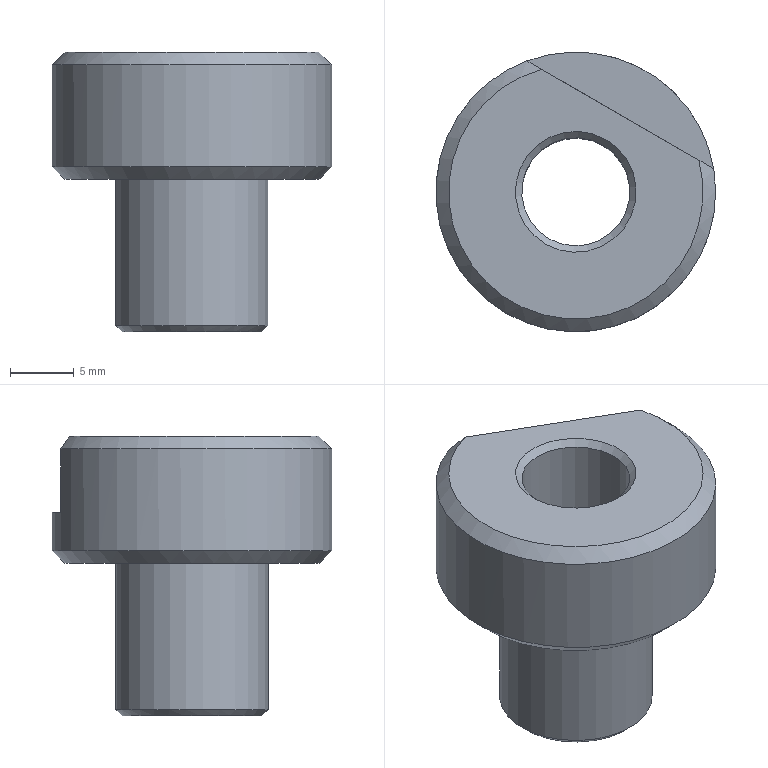Component | NX | DRILL_BUSH_5 | 1 solid | 13 faces | box 22 x 22 x 22 mm | volume 3557 mm3 | plane 5 | cone 5 | cylinder 3 | commonest cylinder face diameters 12 x1 22 x1 8.5 x1
STEP:
#1=CARTESIAN_POINT('',(0.,0.,0.));
#2=DIRECTION('',(0.,0.,1.));
#3=DIRECTION('',(1.,0.,0.));
#4=AXIS2_PLACEMENT_3D('',#1,#2,#3);
#5=CARTESIAN_POINT('',(-32.75,-56.725,158.));
#6=VERTEX_POINT('',#5);
#7=CARTESIAN_POINT('',(-30.,-51.962,158.));
#8=DIRECTION('',(0.,0.,-1.));
#9=DIRECTION('',(-0.5,-0.866,0.));
#10=AXIS2_PLACEMENT_3D('',#7,#8,#9);
#11=CIRCLE('',#10,5.5);
#12=CARTESIAN_POINT('',(-30.,-51.962,158.));
#13=DIRECTION('',(0.,0.,-1.));
#14=DIRECTION('',(-0.5,-0.866,0.));
#15=AXIS2_PLACEMENT_3D('',#12,#13,#14);
#16=PLANE('',#15);
#17=CARTESIAN_POINT('',(0.,0.));
#18=DIRECTION('',(1.,0.));
#19=AXIS2_PLACEMENT_2D('',#17,#18);
#20=CIRCLE('',#19,5.5);
#21=(GEOMETRIC_REPRESENTATION_CONTEXT(2)PARAMETRIC_REPRESENTATION_CONTEXT()REPRESENTATION_CONTEXT('',''));
#22=DEFINITIONAL_REPRESENTATION('',(#20),#21);
#23=PCURVE('',#16,#22);
#24=CARTESIAN_POINT('',(-30.,-51.962,158.5));
#25=DIRECTION('',(0.,0.,1.));
#26=DIRECTION('',(0.5,0.866,0.));
#27=AXIS2_PLACEMENT_3D('',#24,#25,#26);
#28=CONICAL_SURFACE('',#27,6.,0.7854);
#29=CARTESIAN_POINT('',(9.425,-0.5));
#30=DIRECTION('',(-1.,0.));
#31=VECTOR('',#30,1.);
#32=LINE('',#29,#31);
#33=(GEOMETRIC_REPRESENTATION_CONTEXT(2)PARAMETRIC_REPRESENTATION_CONTEXT()REPRESENTATION_CONTEXT('',''));
#34=DEFINITIONAL_REPRESENTATION('',(#32),#33);
#35=PCURVE('',#28,#34);
#36=SURFACE_CURVE('',#11,(#23,#35),.PCURVE_S1.);
#37=EDGE_CURVE('',#6,#6,#36,.T.);
#38=ORIENTED_EDGE('',*,*,#37,.T.);
#39=EDGE_LOOP('',(#38));
#40=FACE_BOUND('',#39,.T.);
#41=CARTESIAN_POINT('',(-32.375,-56.075,158.));
#42=VERTEX_POINT('',#41);
#43=CARTESIAN_POINT('',(-30.,-51.962,158.));
#44=DIRECTION('',(0.,0.,1.));
#45=DIRECTION('',(-0.5,-0.866,0.));
#46=AXIS2_PLACEMENT_3D('',#43,#44,#45);
#47=CIRCLE('',#46,4.75);
#48=CARTESIAN_POINT('',(4.75,0.));
#49=CARTESIAN_POINT('',(4.75,-8.227));
#50=CARTESIAN_POINT('',(-2.375,-4.114));
#51=CARTESIAN_POINT('',(-9.5,-0.));
#52=CARTESIAN_POINT('',(-2.375,4.114));
#53=CARTESIAN_POINT('',(4.75,8.227));
#54=CARTESIAN_POINT('',(4.75,0.));
#55=(BOUNDED_CURVE()B_SPLINE_CURVE(2,(#48,#49,#50,#51,#52,#53,#54),.UNSPECIFIED.,.T.,.F.)B_SPLINE_CURVE_WITH_KNOTS((1,2,2,2,2,1),(-2.094,0.,2.094,4.189,6.283,8.378),.UNSPECIFIED.)CURVE()GEOMETRIC_REPRESENTATION_ITEM()RATIONAL_B_SPLINE_CURVE((1.,0.5,1.,0.5,1.,0.5,1.))REPRESENTATION_ITEM(''));
#56=(GEOMETRIC_REPRESENTATION_CONTEXT(2)PARAMETRIC_REPRESENTATION_CONTEXT()REPRESENTATION_CONTEXT('',''));
#57=DEFINITIONAL_REPRESENTATION('',(#55),#56);
#58=PCURVE('',#16,#57);
#59=CARTESIAN_POINT('',(-30.,-51.962,158.5));
#60=DIRECTION('',(0.,0.,-1.));
#61=DIRECTION('',(-0.5,-0.866,0.));
#62=AXIS2_PLACEMENT_3D('',#59,#60,#61);
#63=CONICAL_SURFACE('',#62,4.25,0.7854);
#64=CARTESIAN_POINT('',(6.283,0.5));
#65=DIRECTION('',(-1.,0.));
#66=VECTOR('',#65,1.);
#67=LINE('',#64,#66);
#68=(GEOMETRIC_REPRESENTATION_CONTEXT(2)PARAMETRIC_REPRESENTATION_CONTEXT()REPRESENTATION_CONTEXT('',''));
#69=DEFINITIONAL_REPRESENTATION('',(#67),#68);
#70=PCURVE('',#63,#69);
#71=SURFACE_CURVE('',#47,(#58,#70),.PCURVE_S1.);
#72=EDGE_CURVE('',#42,#42,#71,.T.);
#73=ORIENTED_EDGE('',*,*,#72,.T.);
#74=EDGE_LOOP('',(#73));
#75=FACE_BOUND('',#74,.T.);
#76=ADVANCED_FACE('',(#40,#75),#16,.T.);
#77=CARTESIAN_POINT('',(-33.,-57.158,158.5));
#78=VERTEX_POINT('',#77);
#79=CARTESIAN_POINT('',(-30.,-51.962,158.5));
#80=DIRECTION('',(0.,0.,1.));
#81=DIRECTION('',(-0.5,-0.866,0.));
#82=AXIS2_PLACEMENT_3D('',#79,#80,#81);
#83=CIRCLE('',#82,6.);
#84=CARTESIAN_POINT('',(-30.,-51.962,158.));
#85=DIRECTION('',(0.,0.,1.));
#86=DIRECTION('',(0.5,0.866,0.));
#87=AXIS2_PLACEMENT_3D('',#84,#85,#86);
#88=CYLINDRICAL_SURFACE('',#87,6.);
#89=CARTESIAN_POINT('',(3.142,0.5));
#90=DIRECTION('',(1.,0.));
#91=VECTOR('',#90,1.);
#92=LINE('',#89,#91);
#93=(GEOMETRIC_REPRESENTATION_CONTEXT(2)PARAMETRIC_REPRESENTATION_CONTEXT()REPRESENTATION_CONTEXT('',''));
#94=DEFINITIONAL_REPRESENTATION('',(#92),#93);
#95=PCURVE('',#88,#94);
#96=CARTESIAN_POINT('',(3.142,-0.));
#97=DIRECTION('',(1.,0.));
#98=VECTOR('',#97,1.);
#99=LINE('',#96,#98);
#100=(GEOMETRIC_REPRESENTATION_CONTEXT(2)PARAMETRIC_REPRESENTATION_CONTEXT()REPRESENTATION_CONTEXT('',''));
#101=DEFINITIONAL_REPRESENTATION('',(#99),#100);
#102=PCURVE('',#28,#101);
#103=SURFACE_CURVE('',#83,(#95,#102),.PCURVE_S1.);
#104=EDGE_CURVE('',#78,#78,#103,.T.);
#105=ORIENTED_EDGE('',*,*,#104,.T.);
#106=CARTESIAN_POINT('',(-33.,-57.158,170.));
#107=VERTEX_POINT('',#106);
#108=CARTESIAN_POINT('',(-33.,-57.158,158.5));
#109=CARTESIAN_POINT('',(-33.,-57.158,170.));
#110=B_SPLINE_CURVE_WITH_KNOTS('',1,(#108,#109),.UNSPECIFIED.,.F.,.F.,(2,2),(0.5,12.),.PIECEWISE_BEZIER_KNOTS.);
#111=CARTESIAN_POINT('',(9.425,0.));
#112=DIRECTION('',(0.,1.));
#113=VECTOR('',#112,1.);
#114=LINE('',#111,#113);
#115=(GEOMETRIC_REPRESENTATION_CONTEXT(2)PARAMETRIC_REPRESENTATION_CONTEXT()REPRESENTATION_CONTEXT('',''));
#116=DEFINITIONAL_REPRESENTATION('',(#114),#115);
#117=PCURVE('',#88,#116);
#118=CARTESIAN_POINT('',(3.142,0.));
#119=DIRECTION('',(0.,1.));
#120=VECTOR('',#119,1.);
#121=LINE('',#118,#120);
#122=(GEOMETRIC_REPRESENTATION_CONTEXT(2)PARAMETRIC_REPRESENTATION_CONTEXT()REPRESENTATION_CONTEXT('',''));
#123=DEFINITIONAL_REPRESENTATION('',(#121),#122);
#124=PCURVE('',#88,#123);
#125=SEAM_CURVE('',#110,(#117,#124),.PCURVE_S1.);
#126=EDGE_CURVE('',#78,#107,#125,.T.);
#127=ORIENTED_EDGE('',*,*,#126,.T.);
#128=CARTESIAN_POINT('',(-30.,-51.962,170.));
#129=DIRECTION('',(0.,0.,1.));
#130=DIRECTION('',(-0.5,-0.866,0.));
#131=AXIS2_PLACEMENT_3D('',#128,#129,#130);
#132=CIRCLE('',#131,6.);
#133=CARTESIAN_POINT('',(3.142,12.));
#134=DIRECTION('',(1.,0.));
#135=VECTOR('',#134,1.);
#136=LINE('',#133,#135);
#137=(GEOMETRIC_REPRESENTATION_CONTEXT(2)PARAMETRIC_REPRESENTATION_CONTEXT()REPRESENTATION_CONTEXT('',''));
#138=DEFINITIONAL_REPRESENTATION('',(#136),#137);
#139=PCURVE('',#88,#138);
#140=CARTESIAN_POINT('',(-30.,-51.962,170.));
#141=DIRECTION('',(0.,0.,-1.));
#142=DIRECTION('',(-0.5,-0.866,0.));
#143=AXIS2_PLACEMENT_3D('',#140,#141,#142);
#144=PLANE('',#143);
#145=CARTESIAN_POINT('',(6.,0.));
#146=CARTESIAN_POINT('',(6.,-10.392));
#147=CARTESIAN_POINT('',(-3.,-5.196));
#148=CARTESIAN_POINT('',(-12.,-0.));
#149=CARTESIAN_POINT('',(-3.,5.196));
#150=CARTESIAN_POINT('',(6.,10.392));
#151=CARTESIAN_POINT('',(6.,0.));
#152=(BOUNDED_CURVE()B_SPLINE_CURVE(2,(#145,#146,#147,#148,#149,#150,#151),.UNSPECIFIED.,.T.,.F.)B_SPLINE_CURVE_WITH_KNOTS((1,2,2,2,2,1),(-2.094,0.,2.094,4.189,6.283,8.378),.UNSPECIFIED.)CURVE()GEOMETRIC_REPRESENTATION_ITEM()RATIONAL_B_SPLINE_CURVE((1.,0.5,1.,0.5,1.,0.5,1.))REPRESENTATION_ITEM(''));
#153=(GEOMETRIC_REPRESENTATION_CONTEXT(2)PARAMETRIC_REPRESENTATION_CONTEXT()REPRESENTATION_CONTEXT('',''));
#154=DEFINITIONAL_REPRESENTATION('',(#152),#153);
#155=PCURVE('',#144,#154);
#156=SURFACE_CURVE('',#132,(#139,#155),.PCURVE_S1.);
#157=EDGE_CURVE('',#107,#107,#156,.T.);
#158=ORIENTED_EDGE('',*,*,#157,.F.);
#159=ORIENTED_EDGE('',*,*,#126,.F.);
#160=EDGE_LOOP('',(#105,#127,#158,#159));
#161=FACE_BOUND('',#160,.T.);
#162=ADVANCED_FACE('',(#161),#88,.T.);
#163=CARTESIAN_POINT('',(-27.625,-47.848,180.));
#164=VERTEX_POINT('',#163);
#165=CARTESIAN_POINT('',(-30.,-51.962,180.));
#166=DIRECTION('',(0.,0.,-1.));
#167=DIRECTION('',(0.5,0.866,0.));
#168=AXIS2_PLACEMENT_3D('',#165,#166,#167);
#169=CIRCLE('',#168,4.75);
#170=CARTESIAN_POINT('',(-30.,-51.962,180.));
#171=DIRECTION('',(0.,0.,1.));
#172=DIRECTION('',(0.5,0.866,0.));
#173=AXIS2_PLACEMENT_3D('',#170,#171,#172);
#174=PLANE('',#173);
#175=CARTESIAN_POINT('',(4.75,0.));
#176=CARTESIAN_POINT('',(4.75,-8.227));
#177=CARTESIAN_POINT('',(-2.375,-4.114));
#178=CARTESIAN_POINT('',(-9.5,-0.));
#179=CARTESIAN_POINT('',(-2.375,4.114));
#180=CARTESIAN_POINT('',(4.75,8.227));
#181=CARTESIAN_POINT('',(4.75,0.));
#182=(BOUNDED_CURVE()B_SPLINE_CURVE(2,(#175,#176,#177,#178,#179,#180,#181),.UNSPECIFIED.,.T.,.F.)B_SPLINE_CURVE_WITH_KNOTS((1,2,2,2,2,1),(-2.094,0.,2.094,4.189,6.283,8.378),.UNSPECIFIED.)CURVE()GEOMETRIC_REPRESENTATION_ITEM()RATIONAL_B_SPLINE_CURVE((1.,0.5,1.,0.5,1.,0.5,1.))REPRESENTATION_ITEM(''));
#183=(GEOMETRIC_REPRESENTATION_CONTEXT(2)PARAMETRIC_REPRESENTATION_CONTEXT()REPRESENTATION_CONTEXT('',''));
#184=DEFINITIONAL_REPRESENTATION('',(#182),#183);
#185=PCURVE('',#174,#184);
#186=CARTESIAN_POINT('',(-30.,-51.962,180.));
#187=DIRECTION('',(0.,0.,1.));
#188=DIRECTION('',(0.5,0.866,0.));
#189=AXIS2_PLACEMENT_3D('',#186,#187,#188);
#190=CONICAL_SURFACE('',#189,4.75,0.7854);
#191=CARTESIAN_POINT('',(6.283,0.));
#192=DIRECTION('',(-1.,0.));
#193=VECTOR('',#192,1.);
#194=LINE('',#191,#193);
#195=(GEOMETRIC_REPRESENTATION_CONTEXT(2)PARAMETRIC_REPRESENTATION_CONTEXT()REPRESENTATION_CONTEXT('',''));
#196=DEFINITIONAL_REPRESENTATION('',(#194),#195);
#197=PCURVE('',#190,#196);
#198=SURFACE_CURVE('',#169,(#185,#197),.PCURVE_S1.);
#199=EDGE_CURVE('',#164,#164,#198,.T.);
#200=ORIENTED_EDGE('',*,*,#199,.T.);
#201=EDGE_LOOP('',(#200));
#202=FACE_BOUND('',#201,.T.);
#203=CARTESIAN_POINT('',(-32.685,-42.329,180.));
#204=VERTEX_POINT('',#203);
#205=CARTESIAN_POINT('',(-20.315,-49.47,180.));
#206=VERTEX_POINT('',#205);
#207=CARTESIAN_POINT('',(-37.758,-39.399,180.));
#208=DIRECTION('',(0.866,-0.5,0.));
#209=VECTOR('',#208,1.);
#210=LINE('',#207,#209);
#211=CARTESIAN_POINT('',(7.,13.));
#212=DIRECTION('',(0.,-1.));
#213=VECTOR('',#212,1.);
#214=LINE('',#211,#213);
#215=(GEOMETRIC_REPRESENTATION_CONTEXT(2)PARAMETRIC_REPRESENTATION_CONTEXT()REPRESENTATION_CONTEXT('',''));
#216=DEFINITIONAL_REPRESENTATION('',(#214),#215);
#217=PCURVE('',#174,#216);
#218=CARTESIAN_POINT('',(-37.758,-39.399,174.));
#219=DIRECTION('',(-0.5,-0.866,0.));
#220=DIRECTION('',(0.866,-0.5,0.));
#221=AXIS2_PLACEMENT_3D('',#218,#219,#220);
#222=PLANE('',#221);
#223=CARTESIAN_POINT('',(0.,6.));
#224=DIRECTION('',(1.,0.));
#225=VECTOR('',#224,1.);
#226=LINE('',#223,#225);
#227=(GEOMETRIC_REPRESENTATION_CONTEXT(2)PARAMETRIC_REPRESENTATION_CONTEXT()REPRESENTATION_CONTEXT('',''));
#228=DEFINITIONAL_REPRESENTATION('',(#226),#227);
#229=PCURVE('',#222,#228);
#230=SURFACE_CURVE('',#210,(#217,#229),.PCURVE_S1.);
#231=EDGE_CURVE('',#204,#206,#230,.T.);
#232=ORIENTED_EDGE('',*,*,#231,.F.);
#233=CARTESIAN_POINT('',(-30.,-51.962,180.));
#234=DIRECTION('',(0.,0.,1.));
#235=DIRECTION('',(0.5,0.866,0.));
#236=AXIS2_PLACEMENT_3D('',#233,#234,#235);
#237=CIRCLE('',#236,10.);
#238=CARTESIAN_POINT('',(0.,0.));
#239=DIRECTION('',(1.,0.));
#240=AXIS2_PLACEMENT_2D('',#238,#239);
#241=CIRCLE('',#240,10.);
#242=(GEOMETRIC_REPRESENTATION_CONTEXT(2)PARAMETRIC_REPRESENTATION_CONTEXT()REPRESENTATION_CONTEXT('',''));
#243=DEFINITIONAL_REPRESENTATION('',(#241),#242);
#244=PCURVE('',#174,#243);
#245=CARTESIAN_POINT('',(-30.,-51.962,179.));
#246=DIRECTION('',(0.,0.,-1.));
#247=DIRECTION('',(-0.5,-0.866,0.));
#248=AXIS2_PLACEMENT_3D('',#245,#246,#247);
#249=CONICAL_SURFACE('',#248,11.,0.7854);
#250=CARTESIAN_POINT('',(3.142,-1.));
#251=DIRECTION('',(-1.,0.));
#252=VECTOR('',#251,1.);
#253=LINE('',#250,#252);
#254=(GEOMETRIC_REPRESENTATION_CONTEXT(2)PARAMETRIC_REPRESENTATION_CONTEXT()REPRESENTATION_CONTEXT('',''));
#255=DEFINITIONAL_REPRESENTATION('',(#253),#254);
#256=PCURVE('',#249,#255);
#257=SURFACE_CURVE('',#237,(#244,#256),.PCURVE_S1.);
#258=EDGE_CURVE('',#204,#206,#257,.T.);
#259=ORIENTED_EDGE('',*,*,#258,.T.);
#260=EDGE_LOOP('',(#232,#259));
#261=FACE_BOUND('',#260,.T.);
#262=ADVANCED_FACE('',(#202,#261),#174,.T.);
#263=CARTESIAN_POINT('',(-35.,-60.622,170.));
#264=VERTEX_POINT('',#263);
#265=CARTESIAN_POINT('',(-30.,-51.962,170.));
#266=DIRECTION('',(0.,0.,-1.));
#267=DIRECTION('',(-0.5,-0.866,0.));
#268=AXIS2_PLACEMENT_3D('',#265,#266,#267);
#269=CIRCLE('',#268,10.);
#270=CARTESIAN_POINT('',(0.,0.));
#271=DIRECTION('',(1.,0.));
#272=AXIS2_PLACEMENT_2D('',#270,#271);
#273=CIRCLE('',#272,10.);
#274=(GEOMETRIC_REPRESENTATION_CONTEXT(2)PARAMETRIC_REPRESENTATION_CONTEXT()REPRESENTATION_CONTEXT('',''));
#275=DEFINITIONAL_REPRESENTATION('',(#273),#274);
#276=PCURVE('',#144,#275);
#277=CARTESIAN_POINT('',(-30.,-51.962,171.));
#278=DIRECTION('',(0.,0.,1.));
#279=DIRECTION('',(0.5,0.866,0.));
#280=AXIS2_PLACEMENT_3D('',#277,#278,#279);
#281=CONICAL_SURFACE('',#280,11.,0.7854);
#282=CARTESIAN_POINT('',(9.425,-1.));
#283=DIRECTION('',(-1.,0.));
#284=VECTOR('',#283,1.);
#285=LINE('',#282,#284);
#286=(GEOMETRIC_REPRESENTATION_CONTEXT(2)PARAMETRIC_REPRESENTATION_CONTEXT()REPRESENTATION_CONTEXT('',''));
#287=DEFINITIONAL_REPRESENTATION('',(#285),#286);
#288=PCURVE('',#281,#287);
#289=SURFACE_CURVE('',#269,(#276,#288),.PCURVE_S1.);
#290=EDGE_CURVE('',#264,#264,#289,.T.);
#291=ORIENTED_EDGE('',*,*,#290,.T.);
#292=EDGE_LOOP('',(#291));
#293=FACE_BOUND('',#292,.T.);
#294=ORIENTED_EDGE('',*,*,#157,.T.);
#295=EDGE_LOOP('',(#294));
#296=FACE_BOUND('',#295,.T.);
#297=ADVANCED_FACE('',(#293,#296),#144,.T.);
#298=CARTESIAN_POINT('',(-35.5,-61.488,171.));
#299=VERTEX_POINT('',#298);
#300=CARTESIAN_POINT('',(-19.152,-50.142,171.));
#301=VERTEX_POINT('',#300);
#302=CARTESIAN_POINT('',(-30.,-51.962,171.));
#303=DIRECTION('',(0.,0.,1.));
#304=DIRECTION('',(-0.5,-0.866,0.));
#305=AXIS2_PLACEMENT_3D('',#302,#303,#304);
#306=CIRCLE('',#305,11.);
#307=CARTESIAN_POINT('',(-30.,-51.962,170.));
#308=DIRECTION('',(0.,0.,1.));
#309=DIRECTION('',(0.5,0.866,0.));
#310=AXIS2_PLACEMENT_3D('',#307,#308,#309);
#311=CYLINDRICAL_SURFACE('',#310,11.);
#312=CARTESIAN_POINT('',(9.425,1.));
#313=DIRECTION('',(1.,0.));
#314=VECTOR('',#313,1.);
#315=LINE('',#312,#314);
#316=(GEOMETRIC_REPRESENTATION_CONTEXT(2)PARAMETRIC_REPRESENTATION_CONTEXT()REPRESENTATION_CONTEXT('',''));
#317=DEFINITIONAL_REPRESENTATION('',(#315),#316);
#318=PCURVE('',#311,#317);
#319=CARTESIAN_POINT('',(3.142,-0.));
#320=DIRECTION('',(1.,0.));
#321=VECTOR('',#320,1.);
#322=LINE('',#319,#321);
#323=(GEOMETRIC_REPRESENTATION_CONTEXT(2)PARAMETRIC_REPRESENTATION_CONTEXT()REPRESENTATION_CONTEXT('',''));
#324=DEFINITIONAL_REPRESENTATION('',(#322),#323);
#325=PCURVE('',#281,#324);
#326=SURFACE_CURVE('',#306,(#318,#325),.PCURVE_S1.);
#327=EDGE_CURVE('',#299,#301,#326,.T.);
#328=ORIENTED_EDGE('',*,*,#327,.T.);
#329=CARTESIAN_POINT('',(-19.152,-50.142,174.));
#330=VERTEX_POINT('',#329);
#331=CARTESIAN_POINT('',(-19.152,-50.142,171.));
#332=CARTESIAN_POINT('',(-19.152,-50.142,174.));
#333=B_SPLINE_CURVE_WITH_KNOTS('',1,(#331,#332),.UNSPECIFIED.,.F.,.F.,(2,2),(1.,4.),.PIECEWISE_BEZIER_KNOTS.);
#334=CARTESIAN_POINT('',(11.685,0.));
#335=DIRECTION('',(0.,1.));
#336=VECTOR('',#335,1.);
#337=LINE('',#334,#336);
#338=(GEOMETRIC_REPRESENTATION_CONTEXT(2)PARAMETRIC_REPRESENTATION_CONTEXT()REPRESENTATION_CONTEXT('',''));
#339=DEFINITIONAL_REPRESENTATION('',(#337),#338);
#340=PCURVE('',#311,#339);
#341=CARTESIAN_POINT('',(5.402,0.));
#342=DIRECTION('',(0.,1.));
#343=VECTOR('',#342,1.);
#344=LINE('',#341,#343);
#345=(GEOMETRIC_REPRESENTATION_CONTEXT(2)PARAMETRIC_REPRESENTATION_CONTEXT()REPRESENTATION_CONTEXT('',''));
#346=DEFINITIONAL_REPRESENTATION('',(#344),#345);
#347=PCURVE('',#311,#346);
#348=SEAM_CURVE('',#333,(#340,#347),.PCURVE_S1.);
#349=EDGE_CURVE('',#301,#330,#348,.T.);
#350=ORIENTED_EDGE('',*,*,#349,.T.);
#351=CARTESIAN_POINT('',(-19.152,-50.142,179.));
#352=VERTEX_POINT('',#351);
#353=CARTESIAN_POINT('',(-19.152,-50.142,170.));
#354=DIRECTION('',(0.,0.,-1.));
#355=VECTOR('',#354,1.);
#356=LINE('',#353,#355);
#357=CARTESIAN_POINT('',(11.685,0.));
#358=DIRECTION('',(0.,-1.));
#359=VECTOR('',#358,1.);
#360=LINE('',#357,#359);
#361=(GEOMETRIC_REPRESENTATION_CONTEXT(2)PARAMETRIC_REPRESENTATION_CONTEXT()REPRESENTATION_CONTEXT('',''));
#362=DEFINITIONAL_REPRESENTATION('',(#360),#361);
#363=PCURVE('',#311,#362);
#364=CARTESIAN_POINT('',(21.485,-4.));
#365=DIRECTION('',(0.,-1.));
#366=VECTOR('',#365,1.);
#367=LINE('',#364,#366);
#368=(GEOMETRIC_REPRESENTATION_CONTEXT(2)PARAMETRIC_REPRESENTATION_CONTEXT()REPRESENTATION_CONTEXT('',''));
#369=DEFINITIONAL_REPRESENTATION('',(#367),#368);
#370=PCURVE('',#222,#369);
#371=SURFACE_CURVE('',#356,(#363,#370),.PCURVE_S1.);
#372=EDGE_CURVE('',#352,#330,#371,.T.);
#373=ORIENTED_EDGE('',*,*,#372,.F.);
#374=CARTESIAN_POINT('',(-33.848,-41.657,179.));
#375=VERTEX_POINT('',#374);
#376=CARTESIAN_POINT('',(-30.,-51.962,179.));
#377=DIRECTION('',(0.,0.,-1.));
#378=DIRECTION('',(0.5,0.866,0.));
#379=AXIS2_PLACEMENT_3D('',#376,#377,#378);
#380=CIRCLE('',#379,11.);
#381=CARTESIAN_POINT('',(12.566,9.));
#382=DIRECTION('',(-1.,0.));
#383=VECTOR('',#382,1.);
#384=LINE('',#381,#383);
#385=(GEOMETRIC_REPRESENTATION_CONTEXT(2)PARAMETRIC_REPRESENTATION_CONTEXT()REPRESENTATION_CONTEXT('',''));
#386=DEFINITIONAL_REPRESENTATION('',(#384),#385);
#387=PCURVE('',#311,#386);
#388=CARTESIAN_POINT('',(-3.142,-0.));
#389=DIRECTION('',(1.,0.));
#390=VECTOR('',#389,1.);
#391=LINE('',#388,#390);
#392=(GEOMETRIC_REPRESENTATION_CONTEXT(2)PARAMETRIC_REPRESENTATION_CONTEXT()REPRESENTATION_CONTEXT('',''));
#393=DEFINITIONAL_REPRESENTATION('',(#391),#392);
#394=PCURVE('',#249,#393);
#395=SURFACE_CURVE('',#380,(#387,#394),.PCURVE_S1.);
#396=EDGE_CURVE('',#352,#375,#395,.T.);
#397=ORIENTED_EDGE('',*,*,#396,.T.);
#398=CARTESIAN_POINT('',(-33.848,-41.657,174.));
#399=VERTEX_POINT('',#398);
#400=CARTESIAN_POINT('',(-33.848,-41.657,170.));
#401=DIRECTION('',(0.,0.,1.));
#402=VECTOR('',#401,1.);
#403=LINE('',#400,#402);
#404=CARTESIAN_POINT('',(7.164,0.));
#405=DIRECTION('',(0.,1.));
#406=VECTOR('',#405,1.);
#407=LINE('',#404,#406);
#408=(GEOMETRIC_REPRESENTATION_CONTEXT(2)PARAMETRIC_REPRESENTATION_CONTEXT()REPRESENTATION_CONTEXT('',''));
#409=DEFINITIONAL_REPRESENTATION('',(#407),#408);
#410=PCURVE('',#311,#409);
#411=CARTESIAN_POINT('',(4.515,-4.));
#412=DIRECTION('',(0.,1.));
#413=VECTOR('',#412,1.);
#414=LINE('',#411,#413);
#415=(GEOMETRIC_REPRESENTATION_CONTEXT(2)PARAMETRIC_REPRESENTATION_CONTEXT()REPRESENTATION_CONTEXT('',''));
#416=DEFINITIONAL_REPRESENTATION('',(#414),#415);
#417=PCURVE('',#222,#416);
#418=SURFACE_CURVE('',#403,(#410,#417),.PCURVE_S1.);
#419=EDGE_CURVE('',#399,#375,#418,.T.);
#420=ORIENTED_EDGE('',*,*,#419,.F.);
#421=CARTESIAN_POINT('',(-30.,-51.962,174.));
#422=DIRECTION('',(0.,0.,-1.));
#423=DIRECTION('',(0.5,0.866,0.));
#424=AXIS2_PLACEMENT_3D('',#421,#422,#423);
#425=CIRCLE('',#424,11.);
#426=CARTESIAN_POINT('',(12.566,4.));
#427=DIRECTION('',(-1.,0.));
#428=VECTOR('',#427,1.);
#429=LINE('',#426,#428);
#430=(GEOMETRIC_REPRESENTATION_CONTEXT(2)PARAMETRIC_REPRESENTATION_CONTEXT()REPRESENTATION_CONTEXT('',''));
#431=DEFINITIONAL_REPRESENTATION('',(#429),#430);
#432=PCURVE('',#311,#431);
#433=CARTESIAN_POINT('',(-30.,-51.962,174.));
#434=DIRECTION('',(0.,0.,1.));
#435=DIRECTION('',(0.5,0.866,0.));
#436=AXIS2_PLACEMENT_3D('',#433,#434,#435);
#437=PLANE('',#436);
#438=CARTESIAN_POINT('',(11.,0.));
#439=CARTESIAN_POINT('',(11.,-19.053));
#440=CARTESIAN_POINT('',(-5.5,-9.526));
#441=CARTESIAN_POINT('',(-22.,-0.));
#442=CARTESIAN_POINT('',(-5.5,9.526));
#443=CARTESIAN_POINT('',(11.,19.053));
#444=CARTESIAN_POINT('',(11.,0.));
#445=(BOUNDED_CURVE()B_SPLINE_CURVE(2,(#438,#439,#440,#441,#442,#443,#444),.UNSPECIFIED.,.T.,.F.)B_SPLINE_CURVE_WITH_KNOTS((1,2,2,2,2,1),(-2.094,0.,2.094,4.189,6.283,8.378),.UNSPECIFIED.)CURVE()GEOMETRIC_REPRESENTATION_ITEM()RATIONAL_B_SPLINE_CURVE((1.,0.5,1.,0.5,1.,0.5,1.))REPRESENTATION_ITEM(''));
#446=(GEOMETRIC_REPRESENTATION_CONTEXT(2)PARAMETRIC_REPRESENTATION_CONTEXT()REPRESENTATION_CONTEXT('',''));
#447=DEFINITIONAL_REPRESENTATION('',(#445),#446);
#448=PCURVE('',#437,#447);
#449=SURFACE_CURVE('',#425,(#432,#448),.PCURVE_S1.);
#450=EDGE_CURVE('',#399,#330,#449,.T.);
#451=ORIENTED_EDGE('',*,*,#450,.T.);
#452=ORIENTED_EDGE('',*,*,#349,.F.);
#453=CARTESIAN_POINT('',(-30.,-51.962,171.));
#454=DIRECTION('',(0.,0.,1.));
#455=DIRECTION('',(-0.5,-0.866,0.));
#456=AXIS2_PLACEMENT_3D('',#453,#454,#455);
#457=CIRCLE('',#456,11.);
#458=CARTESIAN_POINT('',(3.142,1.));
#459=DIRECTION('',(1.,0.));
#460=VECTOR('',#459,1.);
#461=LINE('',#458,#460);
#462=(GEOMETRIC_REPRESENTATION_CONTEXT(2)PARAMETRIC_REPRESENTATION_CONTEXT()REPRESENTATION_CONTEXT('',''));
#463=DEFINITIONAL_REPRESENTATION('',(#461),#462);
#464=PCURVE('',#311,#463);
#465=CARTESIAN_POINT('',(3.142,-0.));
#466=DIRECTION('',(1.,-0.));
#467=VECTOR('',#466,1.);
#468=LINE('',#465,#467);
#469=(GEOMETRIC_REPRESENTATION_CONTEXT(2)PARAMETRIC_REPRESENTATION_CONTEXT()REPRESENTATION_CONTEXT('',''));
#470=DEFINITIONAL_REPRESENTATION('',(#468),#469);
#471=PCURVE('',#281,#470);
#472=SURFACE_CURVE('',#457,(#464,#471),.PCURVE_S1.);
#473=EDGE_CURVE('',#301,#299,#472,.T.);
#474=ORIENTED_EDGE('',*,*,#473,.T.);
#475=EDGE_LOOP('',(#328,#350,#373,#397,#420,#451,#452,#474));
#476=FACE_BOUND('',#475,.T.);
#477=ADVANCED_FACE('',(#476),#311,.T.);
#478=CARTESIAN_POINT('',(-32.125,-55.642,158.5));
#479=VERTEX_POINT('',#478);
#480=CARTESIAN_POINT('',(-30.,-51.962,158.5));
#481=DIRECTION('',(0.,0.,-1.));
#482=DIRECTION('',(-0.5,-0.866,0.));
#483=AXIS2_PLACEMENT_3D('',#480,#481,#482);
#484=CIRCLE('',#483,4.25);
#485=CARTESIAN_POINT('',(-30.,-51.962,180.));
#486=DIRECTION('',(0.,0.,-1.));
#487=DIRECTION('',(-0.5,-0.866,0.));
#488=AXIS2_PLACEMENT_3D('',#485,#486,#487);
#489=CYLINDRICAL_SURFACE('',#488,4.25);
#490=CARTESIAN_POINT('',(0.,21.5));
#491=DIRECTION('',(1.,0.));
#492=VECTOR('',#491,1.);
#493=LINE('',#490,#492);
#494=(GEOMETRIC_REPRESENTATION_CONTEXT(2)PARAMETRIC_REPRESENTATION_CONTEXT()REPRESENTATION_CONTEXT('',''));
#495=DEFINITIONAL_REPRESENTATION('',(#493),#494);
#496=PCURVE('',#489,#495);
#497=CARTESIAN_POINT('',(0.,0.));
#498=DIRECTION('',(1.,0.));
#499=VECTOR('',#498,1.);
#500=LINE('',#497,#499);
#501=(GEOMETRIC_REPRESENTATION_CONTEXT(2)PARAMETRIC_REPRESENTATION_CONTEXT()REPRESENTATION_CONTEXT('',''));
#502=DEFINITIONAL_REPRESENTATION('',(#500),#501);
#503=PCURVE('',#63,#502);
#504=SURFACE_CURVE('',#484,(#496,#503),.PCURVE_S1.);
#505=EDGE_CURVE('',#479,#479,#504,.T.);
#506=ORIENTED_EDGE('',*,*,#505,.F.);
#507=CARTESIAN_POINT('',(-32.125,-55.642,179.5));
#508=VERTEX_POINT('',#507);
#509=CARTESIAN_POINT('',(-32.125,-55.642,179.5));
#510=CARTESIAN_POINT('',(-32.125,-55.642,158.5));
#511=B_SPLINE_CURVE_WITH_KNOTS('',1,(#509,#510),.UNSPECIFIED.,.F.,.F.,(2,2),(0.5,21.5),.PIECEWISE_BEZIER_KNOTS.);
#512=CARTESIAN_POINT('',(0.,0.));
#513=DIRECTION('',(0.,1.));
#514=VECTOR('',#513,1.);
#515=LINE('',#512,#514);
#516=(GEOMETRIC_REPRESENTATION_CONTEXT(2)PARAMETRIC_REPRESENTATION_CONTEXT()REPRESENTATION_CONTEXT('',''));
#517=DEFINITIONAL_REPRESENTATION('',(#515),#516);
#518=PCURVE('',#489,#517);
#519=CARTESIAN_POINT('',(6.283,0.));
#520=DIRECTION('',(0.,1.));
#521=VECTOR('',#520,1.);
#522=LINE('',#519,#521);
#523=(GEOMETRIC_REPRESENTATION_CONTEXT(2)PARAMETRIC_REPRESENTATION_CONTEXT()REPRESENTATION_CONTEXT('',''));
#524=DEFINITIONAL_REPRESENTATION('',(#522),#523);
#525=PCURVE('',#489,#524);
#526=SEAM_CURVE('',#511,(#518,#525),.PCURVE_S1.);
#527=EDGE_CURVE('',#508,#479,#526,.T.);
#528=ORIENTED_EDGE('',*,*,#527,.F.);
#529=CARTESIAN_POINT('',(-27.875,-48.281,179.5));
#530=VERTEX_POINT('',#529);
#531=CARTESIAN_POINT('',(-30.,-51.962,179.5));
#532=DIRECTION('',(0.,0.,1.));
#533=DIRECTION('',(0.5,0.866,0.));
#534=AXIS2_PLACEMENT_3D('',#531,#532,#533);
#535=CIRCLE('',#534,4.25);
#536=CARTESIAN_POINT('',(3.142,0.5));
#537=DIRECTION('',(-1.,0.));
#538=VECTOR('',#537,1.);
#539=LINE('',#536,#538);
#540=(GEOMETRIC_REPRESENTATION_CONTEXT(2)PARAMETRIC_REPRESENTATION_CONTEXT()REPRESENTATION_CONTEXT('',''));
#541=DEFINITIONAL_REPRESENTATION('',(#539),#540);
#542=PCURVE('',#489,#541);
#543=CARTESIAN_POINT('',(0.,-0.5));
#544=DIRECTION('',(1.,0.));
#545=VECTOR('',#544,1.);
#546=LINE('',#543,#545);
#547=(GEOMETRIC_REPRESENTATION_CONTEXT(2)PARAMETRIC_REPRESENTATION_CONTEXT()REPRESENTATION_CONTEXT('',''));
#548=DEFINITIONAL_REPRESENTATION('',(#546),#547);
#549=PCURVE('',#190,#548);
#550=SURFACE_CURVE('',#535,(#542,#549),.PCURVE_S1.);
#551=EDGE_CURVE('',#530,#508,#550,.T.);
#552=ORIENTED_EDGE('',*,*,#551,.F.);
#553=CARTESIAN_POINT('',(-30.,-51.962,179.5));
#554=DIRECTION('',(0.,0.,1.));
#555=DIRECTION('',(0.5,0.866,0.));
#556=AXIS2_PLACEMENT_3D('',#553,#554,#555);
#557=CIRCLE('',#556,4.25);
#558=CARTESIAN_POINT('',(9.425,0.5));
#559=DIRECTION('',(-1.,0.));
#560=VECTOR('',#559,1.);
#561=LINE('',#558,#560);
#562=(GEOMETRIC_REPRESENTATION_CONTEXT(2)PARAMETRIC_REPRESENTATION_CONTEXT()REPRESENTATION_CONTEXT('',''));
#563=DEFINITIONAL_REPRESENTATION('',(#561),#562);
#564=PCURVE('',#489,#563);
#565=CARTESIAN_POINT('',(0.,-0.5));
#566=DIRECTION('',(1.,-0.));
#567=VECTOR('',#566,1.);
#568=LINE('',#565,#567);
#569=(GEOMETRIC_REPRESENTATION_CONTEXT(2)PARAMETRIC_REPRESENTATION_CONTEXT()REPRESENTATION_CONTEXT('',''));
#570=DEFINITIONAL_REPRESENTATION('',(#568),#569);
#571=PCURVE('',#190,#570);
#572=SURFACE_CURVE('',#557,(#564,#571),.PCURVE_S1.);
#573=EDGE_CURVE('',#508,#530,#572,.T.);
#574=ORIENTED_EDGE('',*,*,#573,.F.);
#575=ORIENTED_EDGE('',*,*,#527,.T.);
#576=EDGE_LOOP('',(#506,#528,#552,#574,#575));
#577=FACE_BOUND('',#576,.F.);
#578=ADVANCED_FACE('',(#577),#489,.F.);
#579=ORIENTED_EDGE('',*,*,#419,.T.);
#580=CARTESIAN_POINT('',(-33.848,-41.657,179.));
#581=CARTESIAN_POINT('',(-33.466,-41.878,179.341));
#582=CARTESIAN_POINT('',(-33.078,-42.101,179.676));
#583=CARTESIAN_POINT('',(-32.685,-42.329,180.));
#584=B_SPLINE_CURVE_WITH_KNOTS('',3,(#580,#581,#582,#583),.UNSPECIFIED.,.F.,.F.,(4,4),(0.,1.),.PIECEWISE_BEZIER_KNOTS.);
#585=CARTESIAN_POINT('',(4.515,5.));
#586=CARTESIAN_POINT('',(4.957,5.341));
#587=CARTESIAN_POINT('',(5.404,5.676));
#588=CARTESIAN_POINT('',(5.859,6.));
#589=B_SPLINE_CURVE_WITH_KNOTS('',3,(#585,#586,#587,#588),.UNSPECIFIED.,.F.,.F.,(4,4),(0.,1.),.PIECEWISE_BEZIER_KNOTS.);
#590=(GEOMETRIC_REPRESENTATION_CONTEXT(2)PARAMETRIC_REPRESENTATION_CONTEXT()REPRESENTATION_CONTEXT('',''));
#591=DEFINITIONAL_REPRESENTATION('',(#589),#590);
#592=PCURVE('',#222,#591);
#593=CARTESIAN_POINT('',(2.261,0.));
#594=CARTESIAN_POINT('',(2.346,-1.));
#595=B_SPLINE_CURVE_WITH_KNOTS('',1,(#593,#594),.UNSPECIFIED.,.F.,.F.,(2,2),(0.,1.),.PIECEWISE_BEZIER_KNOTS.);
#596=(GEOMETRIC_REPRESENTATION_CONTEXT(2)PARAMETRIC_REPRESENTATION_CONTEXT()REPRESENTATION_CONTEXT('',''));
#597=DEFINITIONAL_REPRESENTATION('',(#595),#596);
#598=PCURVE('',#249,#597);
#599=SURFACE_CURVE('',#584,(#592,#598),.PCURVE_S1.);
#600=EDGE_CURVE('',#375,#204,#599,.T.);
#601=ORIENTED_EDGE('',*,*,#600,.T.);
#602=ORIENTED_EDGE('',*,*,#231,.T.);
#603=CARTESIAN_POINT('',(-20.315,-49.47,180.));
#604=CARTESIAN_POINT('',(-19.922,-49.697,179.676));
#605=CARTESIAN_POINT('',(-19.534,-49.921,179.341));
#606=CARTESIAN_POINT('',(-19.152,-50.142,179.));
#607=B_SPLINE_CURVE_WITH_KNOTS('',3,(#603,#604,#605,#606),.UNSPECIFIED.,.F.,.F.,(4,4),(0.,1.),.PIECEWISE_BEZIER_KNOTS.);
#608=CARTESIAN_POINT('',(20.141,6.));
#609=CARTESIAN_POINT('',(20.596,5.676));
#610=CARTESIAN_POINT('',(21.043,5.341));
#611=CARTESIAN_POINT('',(21.485,5.));
#612=B_SPLINE_CURVE_WITH_KNOTS('',3,(#608,#609,#610,#611),.UNSPECIFIED.,.F.,.F.,(4,4),(0.,1.),.PIECEWISE_BEZIER_KNOTS.);
#613=(GEOMETRIC_REPRESENTATION_CONTEXT(2)PARAMETRIC_REPRESENTATION_CONTEXT()REPRESENTATION_CONTEXT('',''));
#614=DEFINITIONAL_REPRESENTATION('',(#612),#613);
#615=PCURVE('',#222,#614);
#616=CARTESIAN_POINT('',(-2.346,-1.));
#617=CARTESIAN_POINT('',(-2.261,-0.));
#618=B_SPLINE_CURVE_WITH_KNOTS('',1,(#616,#617),.UNSPECIFIED.,.F.,.F.,(2,2),(0.,1.),.PIECEWISE_BEZIER_KNOTS.);
#619=(GEOMETRIC_REPRESENTATION_CONTEXT(2)PARAMETRIC_REPRESENTATION_CONTEXT()REPRESENTATION_CONTEXT('',''));
#620=DEFINITIONAL_REPRESENTATION('',(#618),#619);
#621=PCURVE('',#249,#620);
#622=SURFACE_CURVE('',#607,(#615,#621),.PCURVE_S1.);
#623=EDGE_CURVE('',#206,#352,#622,.T.);
#624=ORIENTED_EDGE('',*,*,#623,.T.);
#625=ORIENTED_EDGE('',*,*,#372,.T.);
#626=CARTESIAN_POINT('',(-37.758,-39.399,174.));
#627=DIRECTION('',(-0.866,0.5,0.));
#628=VECTOR('',#627,1.);
#629=LINE('',#626,#628);
#630=CARTESIAN_POINT('',(0.,0.));
#631=DIRECTION('',(-1.,0.));
#632=VECTOR('',#631,1.);
#633=LINE('',#630,#632);
#634=(GEOMETRIC_REPRESENTATION_CONTEXT(2)PARAMETRIC_REPRESENTATION_CONTEXT()REPRESENTATION_CONTEXT('',''));
#635=DEFINITIONAL_REPRESENTATION('',(#633),#634);
#636=PCURVE('',#222,#635);
#637=CARTESIAN_POINT('',(7.,13.));
#638=DIRECTION('',(0.,1.));
#639=VECTOR('',#638,1.);
#640=LINE('',#637,#639);
#641=(GEOMETRIC_REPRESENTATION_CONTEXT(2)PARAMETRIC_REPRESENTATION_CONTEXT()REPRESENTATION_CONTEXT('',''));
#642=DEFINITIONAL_REPRESENTATION('',(#640),#641);
#643=PCURVE('',#437,#642);
#644=SURFACE_CURVE('',#629,(#636,#643),.PCURVE_S1.);
#645=EDGE_CURVE('',#330,#399,#644,.T.);
#646=ORIENTED_EDGE('',*,*,#645,.T.);
#647=EDGE_LOOP('',(#579,#601,#602,#624,#625,#646));
#648=FACE_BOUND('',#647,.T.);
#649=ADVANCED_FACE('',(#648),#222,.F.);
#650=ORIENTED_EDGE('',*,*,#645,.F.);
#651=ORIENTED_EDGE('',*,*,#450,.F.);
#652=EDGE_LOOP('',(#650,#651));
#653=FACE_BOUND('',#652,.T.);
#654=ADVANCED_FACE('',(#653),#437,.T.);
#655=ORIENTED_EDGE('',*,*,#37,.F.);
#656=CARTESIAN_POINT('',(-32.75,-56.725,158.));
#657=CARTESIAN_POINT('',(-33.,-57.158,158.5));
#658=B_SPLINE_CURVE_WITH_KNOTS('',1,(#656,#657),.UNSPECIFIED.,.F.,.F.,(2,2),(-0.7071,-0.),.PIECEWISE_BEZIER_KNOTS.);
#659=CARTESIAN_POINT('',(9.425,0.));
#660=DIRECTION('',(0.,1.));
#661=VECTOR('',#660,1.);
#662=LINE('',#659,#661);
#663=(GEOMETRIC_REPRESENTATION_CONTEXT(2)PARAMETRIC_REPRESENTATION_CONTEXT()REPRESENTATION_CONTEXT('',''));
#664=DEFINITIONAL_REPRESENTATION('',(#662),#663);
#665=PCURVE('',#28,#664);
#666=CARTESIAN_POINT('',(3.142,0.));
#667=DIRECTION('',(0.,1.));
#668=VECTOR('',#667,1.);
#669=LINE('',#666,#668);
#670=(GEOMETRIC_REPRESENTATION_CONTEXT(2)PARAMETRIC_REPRESENTATION_CONTEXT()REPRESENTATION_CONTEXT('',''));
#671=DEFINITIONAL_REPRESENTATION('',(#669),#670);
#672=PCURVE('',#28,#671);
#673=SEAM_CURVE('',#658,(#665,#672),.PCURVE_S1.);
#674=EDGE_CURVE('',#6,#78,#673,.T.);
#675=ORIENTED_EDGE('',*,*,#674,.T.);
#676=ORIENTED_EDGE('',*,*,#104,.F.);
#677=ORIENTED_EDGE('',*,*,#674,.F.);
#678=EDGE_LOOP('',(#655,#675,#676,#677));
#679=FACE_BOUND('',#678,.T.);
#680=ADVANCED_FACE('',(#679),#28,.T.);
#681=ORIENTED_EDGE('',*,*,#72,.T.);
#682=CARTESIAN_POINT('',(-32.125,-55.642,158.5));
#683=CARTESIAN_POINT('',(-32.375,-56.075,158.));
#684=B_SPLINE_CURVE_WITH_KNOTS('',1,(#682,#683),.UNSPECIFIED.,.F.,.F.,(2,2),(0.,0.7071),.PIECEWISE_BEZIER_KNOTS.);
#685=CARTESIAN_POINT('',(0.,0.));
#686=DIRECTION('',(0.,1.));
#687=VECTOR('',#686,1.);
#688=LINE('',#685,#687);
#689=(GEOMETRIC_REPRESENTATION_CONTEXT(2)PARAMETRIC_REPRESENTATION_CONTEXT()REPRESENTATION_CONTEXT('',''));
#690=DEFINITIONAL_REPRESENTATION('',(#688),#689);
#691=PCURVE('',#63,#690);
#692=CARTESIAN_POINT('',(6.283,0.));
#693=DIRECTION('',(0.,1.));
#694=VECTOR('',#693,1.);
#695=LINE('',#692,#694);
#696=(GEOMETRIC_REPRESENTATION_CONTEXT(2)PARAMETRIC_REPRESENTATION_CONTEXT()REPRESENTATION_CONTEXT('',''));
#697=DEFINITIONAL_REPRESENTATION('',(#695),#696);
#698=PCURVE('',#63,#697);
#699=SEAM_CURVE('',#684,(#691,#698),.PCURVE_S1.);
#700=EDGE_CURVE('',#479,#42,#699,.T.);
#701=ORIENTED_EDGE('',*,*,#700,.F.);
#702=ORIENTED_EDGE('',*,*,#505,.T.);
#703=ORIENTED_EDGE('',*,*,#700,.T.);
#704=EDGE_LOOP('',(#681,#701,#702,#703));
#705=FACE_BOUND('',#704,.F.);
#706=ADVANCED_FACE('',(#705),#63,.F.);
#707=ORIENTED_EDGE('',*,*,#573,.T.);
#708=CARTESIAN_POINT('',(-27.875,-48.281,179.5));
#709=CARTESIAN_POINT('',(-27.625,-47.848,180.));
#710=B_SPLINE_CURVE_WITH_KNOTS('',1,(#708,#709),.UNSPECIFIED.,.F.,.F.,(2,2),(-0.7071,0.),.PIECEWISE_BEZIER_KNOTS.);
#711=CARTESIAN_POINT('',(6.283,0.));
#712=DIRECTION('',(0.,1.));
#713=VECTOR('',#712,1.);
#714=LINE('',#711,#713);
#715=(GEOMETRIC_REPRESENTATION_CONTEXT(2)PARAMETRIC_REPRESENTATION_CONTEXT()REPRESENTATION_CONTEXT('',''));
#716=DEFINITIONAL_REPRESENTATION('',(#714),#715);
#717=PCURVE('',#190,#716);
#718=CARTESIAN_POINT('',(0.,0.));
#719=DIRECTION('',(0.,1.));
#720=VECTOR('',#719,1.);
#721=LINE('',#718,#720);
#722=(GEOMETRIC_REPRESENTATION_CONTEXT(2)PARAMETRIC_REPRESENTATION_CONTEXT()REPRESENTATION_CONTEXT('',''));
#723=DEFINITIONAL_REPRESENTATION('',(#721),#722);
#724=PCURVE('',#190,#723);
#725=SEAM_CURVE('',#710,(#717,#724),.PCURVE_S1.);
#726=EDGE_CURVE('',#530,#164,#725,.T.);
#727=ORIENTED_EDGE('',*,*,#726,.T.);
#728=ORIENTED_EDGE('',*,*,#199,.T.);
#729=ORIENTED_EDGE('',*,*,#726,.F.);
#730=ORIENTED_EDGE('',*,*,#551,.T.);
#731=EDGE_LOOP('',(#707,#727,#728,#729,#730));
#732=FACE_BOUND('',#731,.F.);
#733=ADVANCED_FACE('',(#732),#190,.F.);
#734=ORIENTED_EDGE('',*,*,#290,.F.);
#735=CARTESIAN_POINT('',(-35.,-60.622,170.));
#736=CARTESIAN_POINT('',(-35.5,-61.488,171.));
#737=B_SPLINE_CURVE_WITH_KNOTS('',1,(#735,#736),.UNSPECIFIED.,.F.,.F.,(2,2),(-1.414,-0.),.PIECEWISE_BEZIER_KNOTS.);
#738=CARTESIAN_POINT('',(9.425,0.));
#739=DIRECTION('',(0.,1.));
#740=VECTOR('',#739,1.);
#741=LINE('',#738,#740);
#742=(GEOMETRIC_REPRESENTATION_CONTEXT(2)PARAMETRIC_REPRESENTATION_CONTEXT()REPRESENTATION_CONTEXT('',''));
#743=DEFINITIONAL_REPRESENTATION('',(#741),#742);
#744=PCURVE('',#281,#743);
#745=CARTESIAN_POINT('',(3.142,0.));
#746=DIRECTION('',(0.,1.));
#747=VECTOR('',#746,1.);
#748=LINE('',#745,#747);
#749=(GEOMETRIC_REPRESENTATION_CONTEXT(2)PARAMETRIC_REPRESENTATION_CONTEXT()REPRESENTATION_CONTEXT('',''));
#750=DEFINITIONAL_REPRESENTATION('',(#748),#749);
#751=PCURVE('',#281,#750);
#752=SEAM_CURVE('',#737,(#744,#751),.PCURVE_S1.);
#753=EDGE_CURVE('',#264,#299,#752,.T.);
#754=ORIENTED_EDGE('',*,*,#753,.T.);
#755=ORIENTED_EDGE('',*,*,#473,.F.);
#756=ORIENTED_EDGE('',*,*,#327,.F.);
#757=ORIENTED_EDGE('',*,*,#753,.F.);
#758=EDGE_LOOP('',(#734,#754,#755,#756,#757));
#759=FACE_BOUND('',#758,.T.);
#760=ADVANCED_FACE('',(#759),#281,.T.);
#761=ORIENTED_EDGE('',*,*,#623,.F.);
#762=ORIENTED_EDGE('',*,*,#258,.F.);
#763=ORIENTED_EDGE('',*,*,#600,.F.);
#764=ORIENTED_EDGE('',*,*,#396,.F.);
#765=EDGE_LOOP('',(#761,#762,#763,#764));
#766=FACE_BOUND('',#765,.T.);
#767=ADVANCED_FACE('',(#766),#249,.T.);
#768=CLOSED_SHELL('',(#76,#162,#262,#297,#477,#578,#649,#654,#680,#706,#733,#760,#767));
#769=MANIFOLD_SOLID_BREP('',#768);
#770=(LENGTH_UNIT()NAMED_UNIT(*)SI_UNIT(.MILLI.,.METRE.));
#771=UNCERTAINTY_MEASURE_WITH_UNIT(LENGTH_MEASURE(0.005),#770,'','');
#772=(NAMED_UNIT(*)PLANE_ANGLE_UNIT()SI_UNIT($,.RADIAN.));
#773=(NAMED_UNIT(*)SI_UNIT($,.STERADIAN.)SOLID_ANGLE_UNIT());
#774=(GEOMETRIC_REPRESENTATION_CONTEXT(3)GLOBAL_UNCERTAINTY_ASSIGNED_CONTEXT((#771))GLOBAL_UNIT_ASSIGNED_CONTEXT((#770,#772,#773))REPRESENTATION_CONTEXT('',''));
#775=ADVANCED_BREP_SHAPE_REPRESENTATION('',(#4,#769),#774);